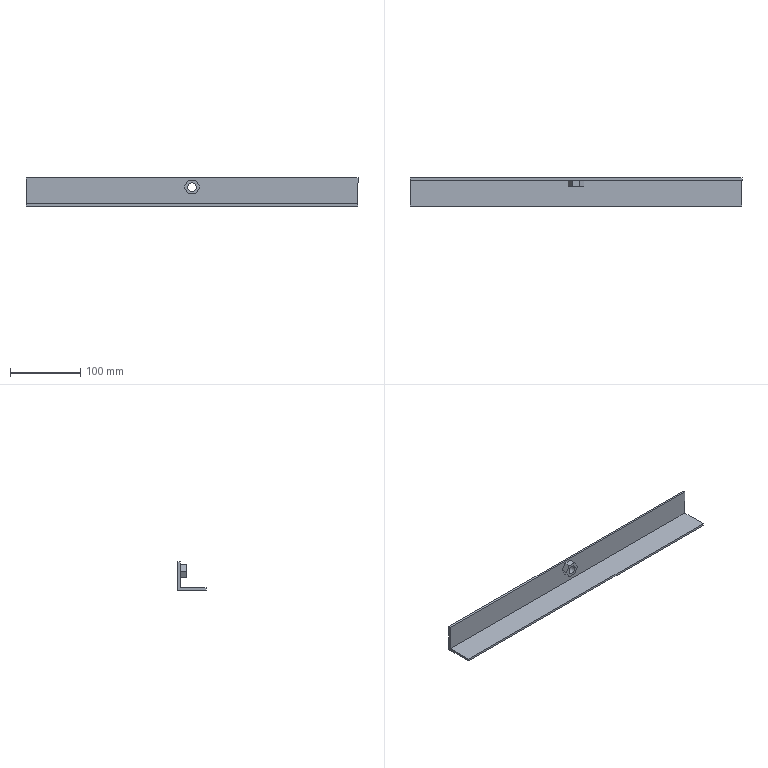Component | SolidWorks | CabinetWelding-1_TopReinforcementAngleIron-1 | 1 solid | 20 faces | box 474 x 40 x 40 mm | volume 110828 mm3 | plane 16 | cylinder 4 | commonest cylinder face diameters 12 x2 14 x2
build123d program:
from build123d import *

# Parameters (mm, degrees)
BOSS_EXTRUDE1_DEPTH = 474
SKETCH2_R           = 7
CUT_EXTRUDE1_DEPTH  = 477
SKETCH3_R           = 6
BOSS_EXTRUDE2_DEPTH = 9


with BuildPart() as part:
    # Sketch1 → Boss-Extrude1 (new body)
    with BuildSketch(Plane.XY):
        Polygon((-34.762, 61.205), (-34.762, 21.205), (-31.762, 21.205), (-31.762, 58.205), (5.238, 58.205), (5.238, 61.205), align=None)
    extrude(amount=BOSS_EXTRUDE1_DEPTH)

    # Sketch2 → Cut-Extrude1 (cut)
    with BuildSketch(Plane(origin=(0, 61.205, 0), x_dir=(1, 0, 0), z_dir=(0, 1, 0))):
        with Locations(Location((-7.762, -237, 0), (0, 0, 270))):
            Circle(SKETCH2_R)
    extrude(amount=-CUT_EXTRUDE1_DEPTH, mode=Mode.SUBTRACT)

    # Sketch3 → Boss-Extrude2 (add)
    with BuildSketch(Plane.XZ.offset(-58.205)):
        Polygon((-7.762, 247.97), (-17.262, 242.485), (-17.262, 231.515), (-7.762, 226.03), (1.738, 231.515), (1.738, 242.485), align=None)
        with Locations(Location((-7.762, 237, 0), (0, 0, 270))):
            Circle(SKETCH3_R, mode=Mode.SUBTRACT)
    extrude(amount=BOSS_EXTRUDE2_DEPTH)


solid = part.part

# Placed as in the assembly
solid = solid.moved(Location((584.082, 830.668, 1385.968), (0, -90, 0)))
STEP:
#1=COLOUR_RGB('',0.7922,0.8196,0.9333);
#2=FILL_AREA_STYLE_COLOUR('',#1);
#3=FILL_AREA_STYLE('',(#2));
#4=SURFACE_STYLE_FILL_AREA(#3);
#5=SURFACE_SIDE_STYLE('',(#4));
#6=SURFACE_STYLE_USAGE(.BOTH.,#5);
#7=PRESENTATION_STYLE_ASSIGNMENT((#6));
#8=CARTESIAN_POINT('',(13.428,34.641,54.26));
#9=VERTEX_POINT('',#8);
#10=CARTESIAN_POINT('',(13.901,34.641,54.26));
#11=VERTEX_POINT('',#10);
#12=CARTESIAN_POINT('',(13.665,34.641,54.26));
#13=DIRECTION('',(-0.,-1.,-0.));
#14=DIRECTION('',(1.,0.,0.));
#15=AXIS2_PLACEMENT_3D('',#12,#13,#14);
#16=CIRCLE('',#15,0.2362);
#17=EDGE_CURVE('',#9,#11,#16,.T.);
#18=ORIENTED_EDGE('',*,*,#17,.T.);
#19=CARTESIAN_POINT('',(13.901,34.995,54.26));
#20=VERTEX_POINT('',#19);
#21=CARTESIAN_POINT('',(13.901,34.641,54.26));
#22=DIRECTION('',(0.,1.,0.));
#23=VECTOR('',#22,39.37);
#24=LINE('',#21,#23);
#25=EDGE_CURVE('',#11,#20,#24,.T.);
#26=ORIENTED_EDGE('',*,*,#25,.T.);
#27=CARTESIAN_POINT('',(13.428,34.995,54.26));
#28=VERTEX_POINT('',#27);
#29=CARTESIAN_POINT('',(13.665,34.995,54.26));
#30=DIRECTION('',(-0.,-1.,-0.));
#31=DIRECTION('',(1.,0.,0.));
#32=AXIS2_PLACEMENT_3D('',#29,#30,#31);
#33=CIRCLE('',#32,0.2362);
#34=EDGE_CURVE('',#28,#20,#33,.T.);
#35=ORIENTED_EDGE('',*,*,#34,.F.);
#36=CARTESIAN_POINT('',(13.428,34.641,54.26));
#37=DIRECTION('',(0.,1.,0.));
#38=VECTOR('',#37,39.37);
#39=LINE('',#36,#38);
#40=EDGE_CURVE('',#9,#28,#39,.T.);
#41=ORIENTED_EDGE('',*,*,#40,.F.);
#42=EDGE_LOOP('',(#18,#26,#35,#41));
#43=FACE_OUTER_BOUND('',#42,.T.);
#44=CARTESIAN_POINT('',(13.665,34.641,54.26));
#45=DIRECTION('',(0.,1.,0.));
#46=DIRECTION('',(-1.,0.,0.));
#47=AXIS2_PLACEMENT_3D('',#44,#45,#46);
#48=CYLINDRICAL_SURFACE('',#47,0.2362);
#49=ADVANCED_FACE('',(#43),#48,.F.);
#50=CARTESIAN_POINT('',(13.94,34.995,54.26));
#51=VERTEX_POINT('',#50);
#52=CARTESIAN_POINT('',(13.389,34.995,54.26));
#53=VERTEX_POINT('',#52);
#54=CARTESIAN_POINT('',(13.665,34.995,54.26));
#55=DIRECTION('',(0.,1.,0.));
#56=DIRECTION('',(-1.,0.,0.));
#57=AXIS2_PLACEMENT_3D('',#54,#55,#56);
#58=CIRCLE('',#57,0.2756);
#59=EDGE_CURVE('',#51,#53,#58,.T.);
#60=ORIENTED_EDGE('',*,*,#59,.F.);
#61=CARTESIAN_POINT('',(13.94,35.113,54.26));
#62=VERTEX_POINT('',#61);
#63=CARTESIAN_POINT('',(13.94,16.334,54.26));
#64=DIRECTION('',(0.,1.,0.));
#65=VECTOR('',#64,39.37);
#66=LINE('',#63,#65);
#67=EDGE_CURVE('',#51,#62,#66,.T.);
#68=ORIENTED_EDGE('',*,*,#67,.T.);
#69=CARTESIAN_POINT('',(13.389,35.113,54.26));
#70=VERTEX_POINT('',#69);
#71=CARTESIAN_POINT('',(13.665,35.113,54.26));
#72=DIRECTION('',(0.,1.,0.));
#73=DIRECTION('',(-1.,0.,0.));
#74=AXIS2_PLACEMENT_3D('',#71,#72,#73);
#75=CIRCLE('',#74,0.2756);
#76=EDGE_CURVE('',#62,#70,#75,.T.);
#77=ORIENTED_EDGE('',*,*,#76,.T.);
#78=CARTESIAN_POINT('',(13.389,16.334,54.26));
#79=DIRECTION('',(0.,1.,0.));
#80=VECTOR('',#79,39.37);
#81=LINE('',#78,#80);
#82=EDGE_CURVE('',#53,#70,#81,.T.);
#83=ORIENTED_EDGE('',*,*,#82,.F.);
#84=EDGE_LOOP('',(#60,#68,#77,#83));
#85=FACE_OUTER_BOUND('',#84,.T.);
#86=CARTESIAN_POINT('',(13.665,16.334,54.26));
#87=DIRECTION('',(0.,1.,0.));
#88=DIRECTION('',(-1.,0.,0.));
#89=AXIS2_PLACEMENT_3D('',#86,#87,#88);
#90=CYLINDRICAL_SURFACE('',#89,0.2756);
#91=ADVANCED_FACE('',(#85),#90,.F.);
#92=CARTESIAN_POINT('',(22.995,34.995,53.315));
#93=VERTEX_POINT('',#92);
#94=CARTESIAN_POINT('',(22.995,34.995,54.772));
#95=VERTEX_POINT('',#94);
#96=CARTESIAN_POINT('',(22.995,34.995,53.315));
#97=DIRECTION('',(0.,-0.,1.));
#98=VECTOR('',#97,39.37);
#99=LINE('',#96,#98);
#100=EDGE_CURVE('',#93,#95,#99,.T.);
#101=ORIENTED_EDGE('',*,*,#100,.T.);
#102=CARTESIAN_POINT('',(4.334,34.995,54.772));
#103=VERTEX_POINT('',#102);
#104=CARTESIAN_POINT('',(4.334,34.995,54.772));
#105=DIRECTION('',(1.,-0.,-0.));
#106=VECTOR('',#105,39.37);
#107=LINE('',#104,#106);
#108=EDGE_CURVE('',#103,#95,#107,.T.);
#109=ORIENTED_EDGE('',*,*,#108,.F.);
#110=CARTESIAN_POINT('',(4.334,34.995,53.315));
#111=VERTEX_POINT('',#110);
#112=CARTESIAN_POINT('',(4.334,34.995,53.315));
#113=DIRECTION('',(0.,-0.,1.));
#114=VECTOR('',#113,39.37);
#115=LINE('',#112,#114);
#116=EDGE_CURVE('',#111,#103,#115,.T.);
#117=ORIENTED_EDGE('',*,*,#116,.F.);
#118=CARTESIAN_POINT('',(4.334,34.995,53.315));
#119=DIRECTION('',(1.,-0.,-0.));
#120=VECTOR('',#119,39.37);
#121=LINE('',#118,#120);
#122=EDGE_CURVE('',#111,#93,#121,.T.);
#123=ORIENTED_EDGE('',*,*,#122,.T.);
#124=EDGE_LOOP('',(#101,#109,#117,#123));
#125=FACE_OUTER_BOUND('',#124,.T.);
#126=CARTESIAN_POINT('',(13.449,34.995,54.634));
#127=VERTEX_POINT('',#126);
#128=CARTESIAN_POINT('',(13.233,34.995,54.26));
#129=VERTEX_POINT('',#128);
#130=CARTESIAN_POINT('',(13.449,34.995,54.634));
#131=DIRECTION('',(-0.5,0.,-0.866));
#132=VECTOR('',#131,39.37);
#133=LINE('',#130,#132);
#134=EDGE_CURVE('',#127,#129,#133,.T.);
#135=ORIENTED_EDGE('',*,*,#134,.F.);
#136=CARTESIAN_POINT('',(13.881,34.995,54.634));
#137=VERTEX_POINT('',#136);
#138=CARTESIAN_POINT('',(13.881,34.995,54.634));
#139=DIRECTION('',(-1.,0.,0.));
#140=VECTOR('',#139,39.37);
#141=LINE('',#138,#140);
#142=EDGE_CURVE('',#137,#127,#141,.T.);
#143=ORIENTED_EDGE('',*,*,#142,.F.);
#144=CARTESIAN_POINT('',(14.097,34.995,54.26));
#145=VERTEX_POINT('',#144);
#146=CARTESIAN_POINT('',(14.097,34.995,54.26));
#147=DIRECTION('',(-0.5,-0.,0.866));
#148=VECTOR('',#147,39.37);
#149=LINE('',#146,#148);
#150=EDGE_CURVE('',#145,#137,#149,.T.);
#151=ORIENTED_EDGE('',*,*,#150,.F.);
#152=CARTESIAN_POINT('',(13.881,34.995,53.886));
#153=VERTEX_POINT('',#152);
#154=CARTESIAN_POINT('',(13.881,34.995,53.886));
#155=DIRECTION('',(0.5,-0.,0.866));
#156=VECTOR('',#155,39.37);
#157=LINE('',#154,#156);
#158=EDGE_CURVE('',#153,#145,#157,.T.);
#159=ORIENTED_EDGE('',*,*,#158,.F.);
#160=CARTESIAN_POINT('',(13.449,34.995,53.886));
#161=VERTEX_POINT('',#160);
#162=CARTESIAN_POINT('',(13.449,34.995,53.886));
#163=DIRECTION('',(1.,-0.,-0.));
#164=VECTOR('',#163,39.37);
#165=LINE('',#162,#164);
#166=EDGE_CURVE('',#161,#153,#165,.T.);
#167=ORIENTED_EDGE('',*,*,#166,.F.);
#168=CARTESIAN_POINT('',(13.233,34.995,54.26));
#169=DIRECTION('',(0.5,0.,-0.866));
#170=VECTOR('',#169,39.37);
#171=LINE('',#168,#170);
#172=EDGE_CURVE('',#129,#161,#171,.T.);
#173=ORIENTED_EDGE('',*,*,#172,.F.);
#174=EDGE_LOOP('',(#135,#143,#151,#159,#167,#173));
#175=FACE_BOUND('',#174,.T.);
#176=CARTESIAN_POINT('',(4.334,34.995,53.315));
#177=DIRECTION('',(0.,1.,0.));
#178=DIRECTION('',(-1.,0.,0.));
#179=AXIS2_PLACEMENT_3D('',#176,#177,#178);
#180=PLANE('',#179);
#181=ADVANCED_FACE('',(#125,#175),#180,.F.);
#182=CARTESIAN_POINT('',(13.665,35.113,54.26));
#183=DIRECTION('',(0.,1.,0.));
#184=DIRECTION('',(-1.,0.,0.));
#185=AXIS2_PLACEMENT_3D('',#182,#183,#184);
#186=CIRCLE('',#185,0.2756);
#187=EDGE_CURVE('',#70,#62,#186,.T.);
#188=ORIENTED_EDGE('',*,*,#187,.F.);
#189=ORIENTED_EDGE('',*,*,#76,.F.);
#190=EDGE_LOOP('',(#188,#189));
#191=FACE_BOUND('',#190,.T.);
#192=CARTESIAN_POINT('',(22.995,35.113,54.772));
#193=VERTEX_POINT('',#192);
#194=CARTESIAN_POINT('',(22.995,35.113,53.197));
#195=VERTEX_POINT('',#194);
#196=CARTESIAN_POINT('',(22.995,35.113,53.197));
#197=DIRECTION('',(-0.,0.,-1.));
#198=VECTOR('',#197,39.37);
#199=LINE('',#196,#198);
#200=EDGE_CURVE('',#193,#195,#199,.T.);
#201=ORIENTED_EDGE('',*,*,#200,.T.);
#202=CARTESIAN_POINT('',(4.334,35.113,53.197));
#203=VERTEX_POINT('',#202);
#204=CARTESIAN_POINT('',(4.334,35.113,53.197));
#205=DIRECTION('',(1.,-0.,-0.));
#206=VECTOR('',#205,39.37);
#207=LINE('',#204,#206);
#208=EDGE_CURVE('',#203,#195,#207,.T.);
#209=ORIENTED_EDGE('',*,*,#208,.F.);
#210=CARTESIAN_POINT('',(4.334,35.113,54.772));
#211=VERTEX_POINT('',#210);
#212=CARTESIAN_POINT('',(4.334,35.113,53.197));
#213=DIRECTION('',(-0.,0.,-1.));
#214=VECTOR('',#213,39.37);
#215=LINE('',#212,#214);
#216=EDGE_CURVE('',#211,#203,#215,.T.);
#217=ORIENTED_EDGE('',*,*,#216,.F.);
#218=CARTESIAN_POINT('',(4.334,35.113,54.772));
#219=DIRECTION('',(1.,-0.,-0.));
#220=VECTOR('',#219,39.37);
#221=LINE('',#218,#220);
#222=EDGE_CURVE('',#211,#193,#221,.T.);
#223=ORIENTED_EDGE('',*,*,#222,.T.);
#224=EDGE_LOOP('',(#201,#209,#217,#223));
#225=FACE_OUTER_BOUND('',#224,.T.);
#226=CARTESIAN_POINT('',(4.334,35.113,53.197));
#227=DIRECTION('',(-0.,-1.,-0.));
#228=DIRECTION('',(1.,-0.,-0.));
#229=AXIS2_PLACEMENT_3D('',#226,#227,#228);
#230=PLANE('',#229);
#231=ADVANCED_FACE('',(#191,#225),#230,.F.);
#232=CARTESIAN_POINT('',(22.995,33.538,53.197));
#233=VERTEX_POINT('',#232);
#234=CARTESIAN_POINT('',(22.995,35.113,53.197));
#235=DIRECTION('',(-0.,-1.,-0.));
#236=VECTOR('',#235,39.37);
#237=LINE('',#234,#236);
#238=EDGE_CURVE('',#195,#233,#237,.T.);
#239=ORIENTED_EDGE('',*,*,#238,.T.);
#240=CARTESIAN_POINT('',(4.334,33.538,53.197));
#241=VERTEX_POINT('',#240);
#242=CARTESIAN_POINT('',(4.334,33.538,53.197));
#243=DIRECTION('',(1.,-0.,-0.));
#244=VECTOR('',#243,39.37);
#245=LINE('',#242,#244);
#246=EDGE_CURVE('',#241,#233,#245,.T.);
#247=ORIENTED_EDGE('',*,*,#246,.F.);
#248=CARTESIAN_POINT('',(4.334,35.113,53.197));
#249=DIRECTION('',(-0.,-1.,-0.));
#250=VECTOR('',#249,39.37);
#251=LINE('',#248,#250);
#252=EDGE_CURVE('',#203,#241,#251,.T.);
#253=ORIENTED_EDGE('',*,*,#252,.F.);
#254=ORIENTED_EDGE('',*,*,#208,.T.);
#255=EDGE_LOOP('',(#239,#247,#253,#254));
#256=FACE_OUTER_BOUND('',#255,.T.);
#257=CARTESIAN_POINT('',(4.334,35.113,53.197));
#258=DIRECTION('',(0.,-0.,1.));
#259=DIRECTION('',(0.,1.,0.));
#260=AXIS2_PLACEMENT_3D('',#257,#258,#259);
#261=PLANE('',#260);
#262=ADVANCED_FACE('',(#256),#261,.F.);
#263=CARTESIAN_POINT('',(22.995,33.538,53.315));
#264=VERTEX_POINT('',#263);
#265=CARTESIAN_POINT('',(22.995,33.538,53.197));
#266=DIRECTION('',(0.,-0.,1.));
#267=VECTOR('',#266,39.37);
#268=LINE('',#265,#267);
#269=EDGE_CURVE('',#233,#264,#268,.T.);
#270=ORIENTED_EDGE('',*,*,#269,.T.);
#271=CARTESIAN_POINT('',(4.334,33.538,53.315));
#272=VERTEX_POINT('',#271);
#273=CARTESIAN_POINT('',(4.334,33.538,53.315));
#274=DIRECTION('',(1.,-0.,-0.));
#275=VECTOR('',#274,39.37);
#276=LINE('',#273,#275);
#277=EDGE_CURVE('',#272,#264,#276,.T.);
#278=ORIENTED_EDGE('',*,*,#277,.F.);
#279=CARTESIAN_POINT('',(4.334,33.538,53.197));
#280=DIRECTION('',(0.,-0.,1.));
#281=VECTOR('',#280,39.37);
#282=LINE('',#279,#281);
#283=EDGE_CURVE('',#241,#272,#282,.T.);
#284=ORIENTED_EDGE('',*,*,#283,.F.);
#285=ORIENTED_EDGE('',*,*,#246,.T.);
#286=EDGE_LOOP('',(#270,#278,#284,#285));
#287=FACE_OUTER_BOUND('',#286,.T.);
#288=CARTESIAN_POINT('',(4.334,33.538,53.197));
#289=DIRECTION('',(0.,1.,0.));
#290=DIRECTION('',(-1.,0.,0.));
#291=AXIS2_PLACEMENT_3D('',#288,#289,#290);
#292=PLANE('',#291);
#293=ADVANCED_FACE('',(#287),#292,.F.);
#294=CARTESIAN_POINT('',(22.995,34.995,53.315));
#295=DIRECTION('',(0.,1.,0.));
#296=VECTOR('',#295,39.37);
#297=LINE('',#294,#296);
#298=EDGE_CURVE('',#264,#93,#297,.T.);
#299=ORIENTED_EDGE('',*,*,#298,.T.);
#300=ORIENTED_EDGE('',*,*,#122,.F.);
#301=CARTESIAN_POINT('',(4.334,34.995,53.315));
#302=DIRECTION('',(0.,1.,0.));
#303=VECTOR('',#302,39.37);
#304=LINE('',#301,#303);
#305=EDGE_CURVE('',#272,#111,#304,.T.);
#306=ORIENTED_EDGE('',*,*,#305,.F.);
#307=ORIENTED_EDGE('',*,*,#277,.T.);
#308=EDGE_LOOP('',(#299,#300,#306,#307));
#309=FACE_OUTER_BOUND('',#308,.T.);
#310=CARTESIAN_POINT('',(4.334,34.995,53.315));
#311=DIRECTION('',(-0.,0.,-1.));
#312=DIRECTION('',(-1.,0.,0.));
#313=AXIS2_PLACEMENT_3D('',#310,#311,#312);
#314=PLANE('',#313);
#315=ADVANCED_FACE('',(#309),#314,.F.);
#316=CARTESIAN_POINT('',(22.995,35.113,54.772));
#317=DIRECTION('',(0.,1.,0.));
#318=VECTOR('',#317,39.37);
#319=LINE('',#316,#318);
#320=EDGE_CURVE('',#95,#193,#319,.T.);
#321=ORIENTED_EDGE('',*,*,#320,.T.);
#322=ORIENTED_EDGE('',*,*,#222,.F.);
#323=CARTESIAN_POINT('',(4.334,35.113,54.772));
#324=DIRECTION('',(0.,1.,0.));
#325=VECTOR('',#324,39.37);
#326=LINE('',#323,#325);
#327=EDGE_CURVE('',#103,#211,#326,.T.);
#328=ORIENTED_EDGE('',*,*,#327,.F.);
#329=ORIENTED_EDGE('',*,*,#108,.T.);
#330=EDGE_LOOP('',(#321,#322,#328,#329));
#331=FACE_OUTER_BOUND('',#330,.T.);
#332=CARTESIAN_POINT('',(4.334,35.113,54.772));
#333=DIRECTION('',(-0.,0.,-1.));
#334=DIRECTION('',(-1.,0.,0.));
#335=AXIS2_PLACEMENT_3D('',#332,#333,#334);
#336=PLANE('',#335);
#337=ADVANCED_FACE('',(#331),#336,.F.);
#338=ORIENTED_EDGE('',*,*,#216,.T.);
#339=ORIENTED_EDGE('',*,*,#252,.T.);
#340=ORIENTED_EDGE('',*,*,#283,.T.);
#341=ORIENTED_EDGE('',*,*,#305,.T.);
#342=ORIENTED_EDGE('',*,*,#116,.T.);
#343=ORIENTED_EDGE('',*,*,#327,.T.);
#344=EDGE_LOOP('',(#338,#339,#340,#341,#342,#343));
#345=FACE_OUTER_BOUND('',#344,.T.);
#346=CARTESIAN_POINT('',(4.334,32.703,54.566));
#347=DIRECTION('',(1.,-0.,-0.));
#348=DIRECTION('',(-0.,0.,-1.));
#349=AXIS2_PLACEMENT_3D('',#346,#347,#348);
#350=PLANE('',#349);
#351=ADVANCED_FACE('',(#345),#350,.F.);
#352=ORIENTED_EDGE('',*,*,#200,.F.);
#353=ORIENTED_EDGE('',*,*,#320,.F.);
#354=ORIENTED_EDGE('',*,*,#100,.F.);
#355=ORIENTED_EDGE('',*,*,#298,.F.);
#356=ORIENTED_EDGE('',*,*,#269,.F.);
#357=ORIENTED_EDGE('',*,*,#238,.F.);
#358=EDGE_LOOP('',(#352,#353,#354,#355,#356,#357));
#359=FACE_OUTER_BOUND('',#358,.T.);
#360=CARTESIAN_POINT('',(22.995,32.703,54.566));
#361=DIRECTION('',(1.,-0.,-0.));
#362=DIRECTION('',(-0.,0.,-1.));
#363=AXIS2_PLACEMENT_3D('',#360,#361,#362);
#364=PLANE('',#363);
#365=ADVANCED_FACE('',(#359),#364,.T.);
#366=ORIENTED_EDGE('',*,*,#67,.F.);
#367=CARTESIAN_POINT('',(13.665,34.995,54.26));
#368=DIRECTION('',(0.,1.,0.));
#369=DIRECTION('',(-1.,0.,0.));
#370=AXIS2_PLACEMENT_3D('',#367,#368,#369);
#371=CIRCLE('',#370,0.2756);
#372=EDGE_CURVE('',#53,#51,#371,.T.);
#373=ORIENTED_EDGE('',*,*,#372,.F.);
#374=ORIENTED_EDGE('',*,*,#82,.T.);
#375=ORIENTED_EDGE('',*,*,#187,.T.);
#376=EDGE_LOOP('',(#366,#373,#374,#375));
#377=FACE_OUTER_BOUND('',#376,.T.);
#378=CARTESIAN_POINT('',(13.665,16.334,54.26));
#379=DIRECTION('',(0.,1.,0.));
#380=DIRECTION('',(-1.,0.,0.));
#381=AXIS2_PLACEMENT_3D('',#378,#379,#380);
#382=CYLINDRICAL_SURFACE('',#381,0.2756);
#383=ADVANCED_FACE('',(#377),#382,.F.);
#384=ORIENTED_EDGE('',*,*,#34,.T.);
#385=CARTESIAN_POINT('',(13.665,34.995,54.26));
#386=DIRECTION('',(-0.,-1.,-0.));
#387=DIRECTION('',(1.,0.,0.));
#388=AXIS2_PLACEMENT_3D('',#385,#386,#387);
#389=CIRCLE('',#388,0.2362);
#390=EDGE_CURVE('',#20,#28,#389,.T.);
#391=ORIENTED_EDGE('',*,*,#390,.T.);
#392=EDGE_LOOP('',(#384,#391));
#393=FACE_BOUND('',#392,.T.);
#394=ORIENTED_EDGE('',*,*,#372,.T.);
#395=ORIENTED_EDGE('',*,*,#59,.T.);
#396=EDGE_LOOP('',(#394,#395));
#397=FACE_OUTER_BOUND('',#396,.T.);
#398=CARTESIAN_POINT('',(22.995,34.995,54.566));
#399=DIRECTION('',(-0.,-1.,-0.));
#400=DIRECTION('',(1.,-0.,-0.));
#401=AXIS2_PLACEMENT_3D('',#398,#399,#400);
#402=PLANE('',#401);
#403=ADVANCED_FACE('',(#393,#397),#402,.F.);
#404=CARTESIAN_POINT('',(13.449,34.641,54.634));
#405=VERTEX_POINT('',#404);
#406=CARTESIAN_POINT('',(13.233,34.641,54.26));
#407=VERTEX_POINT('',#406);
#408=CARTESIAN_POINT('',(13.449,34.641,54.634));
#409=DIRECTION('',(-0.5,0.,-0.866));
#410=VECTOR('',#409,39.37);
#411=LINE('',#408,#410);
#412=EDGE_CURVE('',#405,#407,#411,.T.);
#413=ORIENTED_EDGE('',*,*,#412,.T.);
#414=CARTESIAN_POINT('',(13.449,34.641,53.886));
#415=VERTEX_POINT('',#414);
#416=CARTESIAN_POINT('',(13.233,34.641,54.26));
#417=DIRECTION('',(0.5,0.,-0.866));
#418=VECTOR('',#417,39.37);
#419=LINE('',#416,#418);
#420=EDGE_CURVE('',#407,#415,#419,.T.);
#421=ORIENTED_EDGE('',*,*,#420,.T.);
#422=CARTESIAN_POINT('',(13.881,34.641,53.886));
#423=VERTEX_POINT('',#422);
#424=CARTESIAN_POINT('',(13.449,34.641,53.886));
#425=DIRECTION('',(1.,-0.,-0.));
#426=VECTOR('',#425,39.37);
#427=LINE('',#424,#426);
#428=EDGE_CURVE('',#415,#423,#427,.T.);
#429=ORIENTED_EDGE('',*,*,#428,.T.);
#430=CARTESIAN_POINT('',(14.097,34.641,54.26));
#431=VERTEX_POINT('',#430);
#432=CARTESIAN_POINT('',(13.881,34.641,53.886));
#433=DIRECTION('',(0.5,-0.,0.866));
#434=VECTOR('',#433,39.37);
#435=LINE('',#432,#434);
#436=EDGE_CURVE('',#423,#431,#435,.T.);
#437=ORIENTED_EDGE('',*,*,#436,.T.);
#438=CARTESIAN_POINT('',(13.881,34.641,54.634));
#439=VERTEX_POINT('',#438);
#440=CARTESIAN_POINT('',(14.097,34.641,54.26));
#441=DIRECTION('',(-0.5,-0.,0.866));
#442=VECTOR('',#441,39.37);
#443=LINE('',#440,#442);
#444=EDGE_CURVE('',#431,#439,#443,.T.);
#445=ORIENTED_EDGE('',*,*,#444,.T.);
#446=CARTESIAN_POINT('',(13.881,34.641,54.634));
#447=DIRECTION('',(-1.,0.,0.));
#448=VECTOR('',#447,39.37);
#449=LINE('',#446,#448);
#450=EDGE_CURVE('',#439,#405,#449,.T.);
#451=ORIENTED_EDGE('',*,*,#450,.T.);
#452=EDGE_LOOP('',(#413,#421,#429,#437,#445,#451));
#453=FACE_OUTER_BOUND('',#452,.T.);
#454=ORIENTED_EDGE('',*,*,#17,.F.);
#455=CARTESIAN_POINT('',(13.665,34.641,54.26));
#456=DIRECTION('',(-0.,-1.,-0.));
#457=DIRECTION('',(1.,0.,0.));
#458=AXIS2_PLACEMENT_3D('',#455,#456,#457);
#459=CIRCLE('',#458,0.2362);
#460=EDGE_CURVE('',#11,#9,#459,.T.);
#461=ORIENTED_EDGE('',*,*,#460,.F.);
#462=EDGE_LOOP('',(#454,#461));
#463=FACE_BOUND('',#462,.T.);
#464=CARTESIAN_POINT('',(22.995,34.641,54.566));
#465=DIRECTION('',(-0.,-1.,-0.));
#466=DIRECTION('',(1.,-0.,-0.));
#467=AXIS2_PLACEMENT_3D('',#464,#465,#466);
#468=PLANE('',#467);
#469=ADVANCED_FACE('',(#453,#463),#468,.T.);
#470=ORIENTED_EDGE('',*,*,#134,.T.);
#471=CARTESIAN_POINT('',(13.233,34.641,54.26));
#472=DIRECTION('',(0.,1.,0.));
#473=VECTOR('',#472,39.37);
#474=LINE('',#471,#473);
#475=EDGE_CURVE('',#407,#129,#474,.T.);
#476=ORIENTED_EDGE('',*,*,#475,.F.);
#477=ORIENTED_EDGE('',*,*,#412,.F.);
#478=CARTESIAN_POINT('',(13.449,34.641,54.634));
#479=DIRECTION('',(0.,1.,0.));
#480=VECTOR('',#479,39.37);
#481=LINE('',#478,#480);
#482=EDGE_CURVE('',#405,#127,#481,.T.);
#483=ORIENTED_EDGE('',*,*,#482,.T.);
#484=EDGE_LOOP('',(#470,#476,#477,#483));
#485=FACE_OUTER_BOUND('',#484,.T.);
#486=CARTESIAN_POINT('',(13.449,34.641,54.634));
#487=DIRECTION('',(0.866,-0.,-0.5));
#488=DIRECTION('',(-0.5,0.,-0.866));
#489=AXIS2_PLACEMENT_3D('',#486,#487,#488);
#490=PLANE('',#489);
#491=ADVANCED_FACE('',(#485),#490,.F.);
#492=ORIENTED_EDGE('',*,*,#172,.T.);
#493=CARTESIAN_POINT('',(13.449,34.641,53.886));
#494=DIRECTION('',(0.,1.,0.));
#495=VECTOR('',#494,39.37);
#496=LINE('',#493,#495);
#497=EDGE_CURVE('',#415,#161,#496,.T.);
#498=ORIENTED_EDGE('',*,*,#497,.F.);
#499=ORIENTED_EDGE('',*,*,#420,.F.);
#500=ORIENTED_EDGE('',*,*,#475,.T.);
#501=EDGE_LOOP('',(#492,#498,#499,#500));
#502=FACE_OUTER_BOUND('',#501,.T.);
#503=CARTESIAN_POINT('',(13.233,34.641,54.26));
#504=DIRECTION('',(0.866,-0.,0.5));
#505=DIRECTION('',(0.5,0.,-0.866));
#506=AXIS2_PLACEMENT_3D('',#503,#504,#505);
#507=PLANE('',#506);
#508=ADVANCED_FACE('',(#502),#507,.F.);
#509=ORIENTED_EDGE('',*,*,#166,.T.);
#510=CARTESIAN_POINT('',(13.881,34.641,53.886));
#511=DIRECTION('',(0.,1.,0.));
#512=VECTOR('',#511,39.37);
#513=LINE('',#510,#512);
#514=EDGE_CURVE('',#423,#153,#513,.T.);
#515=ORIENTED_EDGE('',*,*,#514,.F.);
#516=ORIENTED_EDGE('',*,*,#428,.F.);
#517=ORIENTED_EDGE('',*,*,#497,.T.);
#518=EDGE_LOOP('',(#509,#515,#516,#517));
#519=FACE_OUTER_BOUND('',#518,.T.);
#520=CARTESIAN_POINT('',(13.449,34.641,53.886));
#521=DIRECTION('',(0.,-0.,1.));
#522=DIRECTION('',(1.,-0.,-0.));
#523=AXIS2_PLACEMENT_3D('',#520,#521,#522);
#524=PLANE('',#523);
#525=ADVANCED_FACE('',(#519),#524,.F.);
#526=ORIENTED_EDGE('',*,*,#158,.T.);
#527=CARTESIAN_POINT('',(14.097,34.641,54.26));
#528=DIRECTION('',(0.,1.,0.));
#529=VECTOR('',#528,39.37);
#530=LINE('',#527,#529);
#531=EDGE_CURVE('',#431,#145,#530,.T.);
#532=ORIENTED_EDGE('',*,*,#531,.F.);
#533=ORIENTED_EDGE('',*,*,#436,.F.);
#534=ORIENTED_EDGE('',*,*,#514,.T.);
#535=EDGE_LOOP('',(#526,#532,#533,#534));
#536=FACE_OUTER_BOUND('',#535,.T.);
#537=CARTESIAN_POINT('',(13.881,34.641,53.886));
#538=DIRECTION('',(-0.866,0.,0.5));
#539=DIRECTION('',(0.5,-0.,0.866));
#540=AXIS2_PLACEMENT_3D('',#537,#538,#539);
#541=PLANE('',#540);
#542=ADVANCED_FACE('',(#536),#541,.F.);
#543=ORIENTED_EDGE('',*,*,#150,.T.);
#544=CARTESIAN_POINT('',(13.881,34.641,54.634));
#545=DIRECTION('',(0.,1.,0.));
#546=VECTOR('',#545,39.37);
#547=LINE('',#544,#546);
#548=EDGE_CURVE('',#439,#137,#547,.T.);
#549=ORIENTED_EDGE('',*,*,#548,.F.);
#550=ORIENTED_EDGE('',*,*,#444,.F.);
#551=ORIENTED_EDGE('',*,*,#531,.T.);
#552=EDGE_LOOP('',(#543,#549,#550,#551));
#553=FACE_OUTER_BOUND('',#552,.T.);
#554=CARTESIAN_POINT('',(14.097,34.641,54.26));
#555=DIRECTION('',(-0.866,0.,-0.5));
#556=DIRECTION('',(-0.5,-0.,0.866));
#557=AXIS2_PLACEMENT_3D('',#554,#555,#556);
#558=PLANE('',#557);
#559=ADVANCED_FACE('',(#553),#558,.F.);
#560=ORIENTED_EDGE('',*,*,#142,.T.);
#561=ORIENTED_EDGE('',*,*,#482,.F.);
#562=ORIENTED_EDGE('',*,*,#450,.F.);
#563=ORIENTED_EDGE('',*,*,#548,.T.);
#564=EDGE_LOOP('',(#560,#561,#562,#563));
#565=FACE_OUTER_BOUND('',#564,.T.);
#566=CARTESIAN_POINT('',(13.881,34.641,54.634));
#567=DIRECTION('',(-0.,0.,-1.));
#568=DIRECTION('',(-1.,0.,0.));
#569=AXIS2_PLACEMENT_3D('',#566,#567,#568);
#570=PLANE('',#569);
#571=ADVANCED_FACE('',(#565),#570,.F.);
#572=ORIENTED_EDGE('',*,*,#25,.F.);
#573=ORIENTED_EDGE('',*,*,#460,.T.);
#574=ORIENTED_EDGE('',*,*,#40,.T.);
#575=ORIENTED_EDGE('',*,*,#390,.F.);
#576=EDGE_LOOP('',(#572,#573,#574,#575));
#577=FACE_OUTER_BOUND('',#576,.T.);
#578=CARTESIAN_POINT('',(13.665,34.641,54.26));
#579=DIRECTION('',(0.,1.,0.));
#580=DIRECTION('',(-1.,0.,0.));
#581=AXIS2_PLACEMENT_3D('',#578,#579,#580);
#582=CYLINDRICAL_SURFACE('',#581,0.2362);
#583=ADVANCED_FACE('',(#577),#582,.F.);
#584=CLOSED_SHELL('',(#49,#91,#181,#231,#262,#293,#315,#337,#351,#365,#383,#403,#469,#491,#508,#525,#542,#559,#571,#583));
#585=MANIFOLD_SOLID_BREP('',#584);
#586=STYLED_ITEM('',(#7),#585);
#587=PRESENTATION_LAYER_ASSIGNMENT('','',(#586));
#588=CARTESIAN_POINT('',(0.,0.,0.));
#589=DIRECTION('',(0.,0.,1.));
#590=DIRECTION('',(1.,0.,0.));
#591=AXIS2_PLACEMENT_3D('',#588,#589,#590);
#592=(LENGTH_UNIT()NAMED_UNIT(*)SI_UNIT($,.METRE.));
#593=LENGTH_MEASURE_WITH_UNIT(LENGTH_MEASURE(0.0254),#592);
#594=DIMENSIONAL_EXPONENTS(1.,0.,0.,0.,0.,0.,0.);
#595=(CONVERSION_BASED_UNIT('',#593)LENGTH_UNIT()NAMED_UNIT(#594));
#596=UNCERTAINTY_MEASURE_WITH_UNIT(LENGTH_MEASURE(0.00001),#595,'','');
#597=(NAMED_UNIT(*)PLANE_ANGLE_UNIT()SI_UNIT($,.RADIAN.));
#598=(NAMED_UNIT(*)SI_UNIT($,.STERADIAN.)SOLID_ANGLE_UNIT());
#599=(GEOMETRIC_REPRESENTATION_CONTEXT(3)GLOBAL_UNCERTAINTY_ASSIGNED_CONTEXT((#596))GLOBAL_UNIT_ASSIGNED_CONTEXT((#595,#597,#598))REPRESENTATION_CONTEXT('',''));
#600=ADVANCED_BREP_SHAPE_REPRESENTATION('',(#585,#591),#599);
#601=(LENGTH_UNIT()NAMED_UNIT(*)SI_UNIT($,.METRE.));
#602=LENGTH_MEASURE_WITH_UNIT(LENGTH_MEASURE(0.0254),#601);
#603=DIMENSIONAL_EXPONENTS(1.,0.,0.,0.,0.,0.,0.);
#604=(CONVERSION_BASED_UNIT('',#602)LENGTH_UNIT()NAMED_UNIT(#603));
#605=UNCERTAINTY_MEASURE_WITH_UNIT(LENGTH_MEASURE(0.00001),#604,'','');
#606=(NAMED_UNIT(*)PLANE_ANGLE_UNIT()SI_UNIT($,.RADIAN.));
#607=(NAMED_UNIT(*)SI_UNIT($,.STERADIAN.)SOLID_ANGLE_UNIT());
#608=(GEOMETRIC_REPRESENTATION_CONTEXT(3)GLOBAL_UNCERTAINTY_ASSIGNED_CONTEXT((#605))GLOBAL_UNIT_ASSIGNED_CONTEXT((#604,#606,#607))REPRESENTATION_CONTEXT('',''));
#609=MECHANICAL_DESIGN_GEOMETRIC_PRESENTATION_REPRESENTATION('',(#586),#608);